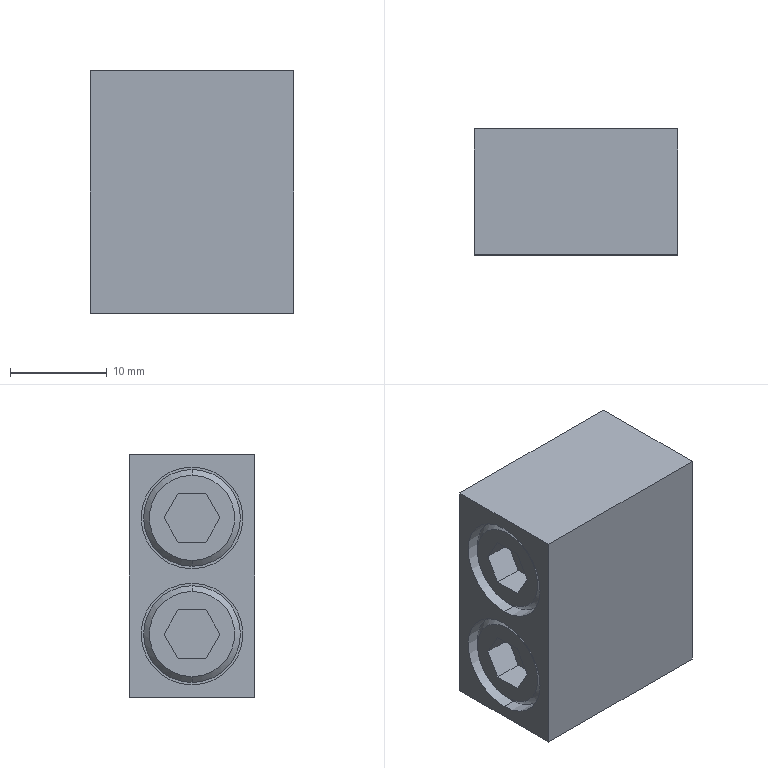Component | SolidWorks | SMC-MXS20-100AS-M9N-1_0SMC-MXS20-100AS-M9N-5-1 | 1 solid | 36 faces | box 21 x 13 x 25 mm | volume 6501 mm3 | plane 24 | cylinder 8 | cone 4 | commonest cylinder face diameters 10 x4 10.5 x4
build123d program:
from build123d import *

# Parameters (mm, degrees)
BOSS_EXTRUDE1_DEPTH      = 6.5
BOSS_EXTRUDE1_DEPTH_BACK = 6.5
SKETCH1_W                = 21
SKETCH1_H                = 25
SKETCH2_R                = 5.25
CUT_EXTRUDE1_DEPTH       = 6.5
SKETCH3_R                = 5.25
CUT_EXTRUDE2_DEPTH       = 6.5
CUT_EXTRUDE3_DEPTH       = 3
CUT_EXTRUDE4_DEPTH       = 3


with BuildPart() as part:
    # Sketch1 → Boss-Extrude1 (new, two sides: drawn at the far end of the back side and taken through both)
    with BuildSketch(Plane(origin=(0, 0, 0), x_dir=(1, 0, 0), z_dir=(0, 1, 0)).offset(-BOSS_EXTRUDE1_DEPTH_BACK)):
        with Locations((-10.5, 0)):
            Rectangle(SKETCH1_W, SKETCH1_H)
    extrude(amount=BOSS_EXTRUDE1_DEPTH + BOSS_EXTRUDE1_DEPTH_BACK)

    # Sketch2 → Cut-Extrude1 (cut)
    with BuildSketch(Plane(origin=(-21, 0, 0), x_dir=(0, 0, -1), z_dir=(1, 0, 0))):
        with Locations((-6, 0)):
            Circle(SKETCH2_R)
    extrude(amount=CUT_EXTRUDE1_DEPTH, mode=Mode.SUBTRACT)

    # Sketch3 → Cut-Extrude2 (cut)
    with BuildSketch(Plane(origin=(-21, 0, 0), x_dir=(0, 0, -1), z_dir=(1, 0, 0))):
        with Locations((6, 0)):
            Circle(SKETCH3_R)
    extrude(amount=CUT_EXTRUDE2_DEPTH, mode=Mode.SUBTRACT)

    # Sketch4 → Revolve1 (revolve)
    with BuildSketch(Plane(origin=(0, 0, 0), x_dir=(1, 0, 0), z_dir=(0, 1, 0)), mode=Mode.PRIVATE) as revolve1_sk:
        Polygon((-14.5, -6), (-14.5, -11), (-19.9, -11), (-20.5, -10.4), (-20.5, -6), align=None)
    revolve(revolve1_sk.sketch.rotate(Axis((-20.5, 0, 6), (1, 0, 0)), 180), axis=Axis((-20.5, 0, 6), (1, 0, 0)))

    # Sketch5 → Revolve2 (revolve)
    with BuildSketch(Plane(origin=(0, 0, 0), x_dir=(1, 0, 0), z_dir=(0, 1, 0)), mode=Mode.PRIVATE) as revolve2_sk:
        Polygon((-14.5, 6), (-14.5, 1), (-19.9, 1), (-20.5, 1.6), (-20.5, 6), align=None)
    revolve(revolve2_sk.sketch.rotate(Axis((-20.5, 0, -6), (1, 0, 0)), 180), axis=Axis((-20.5, 0, -6), (1, 0, 0)))

    # Sketch6 → Cut-Extrude3 (cut)
    with BuildSketch(Plane(origin=(-20.5, 0, 0), x_dir=(0, 0, -1), z_dir=(1, 0, 0))):
        Polygon((-8.5, 1.443), (-8.5, -1.443), (-6, -2.887), (-3.5, -1.443), (-3.5, 1.443), (-6, 2.887), align=None)
    extrude(amount=CUT_EXTRUDE3_DEPTH, mode=Mode.SUBTRACT)

    # Sketch7 → Cut-Extrude4 (cut)
    with BuildSketch(Plane(origin=(-20.5, 0, 0), x_dir=(0, 0, -1), z_dir=(1, 0, 0))):
        Polygon((3.5, 1.443), (3.5, -1.443), (6, -2.887), (8.5, -1.443), (8.5, 1.443), (6, 2.887), align=None)
    extrude(amount=CUT_EXTRUDE4_DEPTH, mode=Mode.SUBTRACT)


solid = part.part

# Placed as in the assembly
solid = solid.moved(Location((-271.009, 86.721, 82.589), (0, 0, 0)))
STEP:
#1=COLOUR_RGB('',0.7922,0.8196,0.9333);
#2=FILL_AREA_STYLE_COLOUR('',#1);
#3=FILL_AREA_STYLE('',(#2));
#4=SURFACE_STYLE_FILL_AREA(#3);
#5=SURFACE_SIDE_STYLE('',(#4));
#6=SURFACE_STYLE_USAGE(.BOTH.,#5);
#7=PRESENTATION_STYLE_ASSIGNMENT((#6));
#8=CARTESIAN_POINT('',(-11.477,3.414,2.842));
#9=VERTEX_POINT('',#8);
#10=CARTESIAN_POINT('',(-11.477,3.414,3.189));
#11=VERTEX_POINT('',#10);
#12=CARTESIAN_POINT('',(-11.477,3.414,3.015));
#13=DIRECTION('',(1.,0.,0.));
#14=DIRECTION('',(0.,0.,-1.));
#15=AXIS2_PLACEMENT_3D('',#12,#13,#14);
#16=CIRCLE('',#15,0.1732);
#17=EDGE_CURVE('',#9,#11,#16,.T.);
#18=ORIENTED_EDGE('',*,*,#17,.T.);
#19=CARTESIAN_POINT('',(-11.453,3.414,3.212));
#20=VERTEX_POINT('',#19);
#21=CARTESIAN_POINT('',(-11.477,3.414,3.189));
#22=DIRECTION('',(0.7071,0.,0.7071));
#23=VECTOR('',#22,39.37);
#24=LINE('',#21,#23);
#25=EDGE_CURVE('',#11,#20,#24,.T.);
#26=ORIENTED_EDGE('',*,*,#25,.T.);
#27=CARTESIAN_POINT('',(-11.453,3.414,2.818));
#28=VERTEX_POINT('',#27);
#29=CARTESIAN_POINT('',(-11.453,3.414,3.015));
#30=DIRECTION('',(1.,0.,0.));
#31=DIRECTION('',(0.,0.,-1.));
#32=AXIS2_PLACEMENT_3D('',#29,#30,#31);
#33=CIRCLE('',#32,0.1969);
#34=EDGE_CURVE('',#28,#20,#33,.T.);
#35=ORIENTED_EDGE('',*,*,#34,.F.);
#36=CARTESIAN_POINT('',(-11.477,3.414,2.842));
#37=DIRECTION('',(0.7071,0.,-0.7071));
#38=VECTOR('',#37,39.37);
#39=LINE('',#36,#38);
#40=EDGE_CURVE('',#9,#28,#39,.T.);
#41=ORIENTED_EDGE('',*,*,#40,.F.);
#42=EDGE_LOOP('',(#18,#26,#35,#41));
#43=FACE_OUTER_BOUND('',#42,.T.);
#44=CARTESIAN_POINT('',(-11.477,3.414,3.015));
#45=DIRECTION('',(1.,0.,0.));
#46=DIRECTION('',(0.,0.,-1.));
#47=AXIS2_PLACEMENT_3D('',#44,#45,#46);
#48=CONICAL_SURFACE('',#47,0.1732,0.7854);
#49=ADVANCED_FACE('',(#43),#48,.T.);
#50=ORIENTED_EDGE('',*,*,#34,.T.);
#51=CARTESIAN_POINT('',(-11.241,3.414,3.212));
#52=VERTEX_POINT('',#51);
#53=CARTESIAN_POINT('',(-11.477,3.414,3.212));
#54=DIRECTION('',(1.,0.,0.));
#55=VECTOR('',#54,39.37);
#56=LINE('',#53,#55);
#57=EDGE_CURVE('',#20,#52,#56,.T.);
#58=ORIENTED_EDGE('',*,*,#57,.T.);
#59=CARTESIAN_POINT('',(-11.241,3.414,2.818));
#60=VERTEX_POINT('',#59);
#61=CARTESIAN_POINT('',(-11.241,3.414,3.015));
#62=DIRECTION('',(-1.,0.,0.));
#63=DIRECTION('',(0.,0.,-1.));
#64=AXIS2_PLACEMENT_3D('',#61,#62,#63);
#65=CIRCLE('',#64,0.1969);
#66=EDGE_CURVE('',#52,#60,#65,.T.);
#67=ORIENTED_EDGE('',*,*,#66,.T.);
#68=CARTESIAN_POINT('',(-11.477,3.414,2.818));
#69=DIRECTION('',(1.,0.,0.));
#70=VECTOR('',#69,39.37);
#71=LINE('',#68,#70);
#72=EDGE_CURVE('',#28,#60,#71,.T.);
#73=ORIENTED_EDGE('',*,*,#72,.F.);
#74=EDGE_LOOP('',(#50,#58,#67,#73));
#75=FACE_OUTER_BOUND('',#74,.T.);
#76=CARTESIAN_POINT('',(-11.477,3.414,3.015));
#77=DIRECTION('',(1.,0.,0.));
#78=DIRECTION('',(0.,0.,-1.));
#79=AXIS2_PLACEMENT_3D('',#76,#77,#78);
#80=CYLINDRICAL_SURFACE('',#79,0.1969);
#81=ADVANCED_FACE('',(#75),#80,.T.);
#82=CARTESIAN_POINT('',(-11.477,3.414,3.315));
#83=VERTEX_POINT('',#82);
#84=CARTESIAN_POINT('',(-11.477,3.414,3.661));
#85=VERTEX_POINT('',#84);
#86=CARTESIAN_POINT('',(-11.477,3.414,3.488));
#87=DIRECTION('',(1.,0.,0.));
#88=DIRECTION('',(0.,0.,-1.));
#89=AXIS2_PLACEMENT_3D('',#86,#87,#88);
#90=CIRCLE('',#89,0.1732);
#91=EDGE_CURVE('',#83,#85,#90,.T.);
#92=ORIENTED_EDGE('',*,*,#91,.T.);
#93=CARTESIAN_POINT('',(-11.453,3.414,3.685));
#94=VERTEX_POINT('',#93);
#95=CARTESIAN_POINT('',(-11.477,3.414,3.661));
#96=DIRECTION('',(0.7071,0.,0.7071));
#97=VECTOR('',#96,39.37);
#98=LINE('',#95,#97);
#99=EDGE_CURVE('',#85,#94,#98,.T.);
#100=ORIENTED_EDGE('',*,*,#99,.T.);
#101=CARTESIAN_POINT('',(-11.453,3.414,3.291));
#102=VERTEX_POINT('',#101);
#103=CARTESIAN_POINT('',(-11.453,3.414,3.488));
#104=DIRECTION('',(1.,0.,0.));
#105=DIRECTION('',(0.,0.,-1.));
#106=AXIS2_PLACEMENT_3D('',#103,#104,#105);
#107=CIRCLE('',#106,0.1969);
#108=EDGE_CURVE('',#102,#94,#107,.T.);
#109=ORIENTED_EDGE('',*,*,#108,.F.);
#110=CARTESIAN_POINT('',(-11.477,3.414,3.315));
#111=DIRECTION('',(0.7071,0.,-0.7071));
#112=VECTOR('',#111,39.37);
#113=LINE('',#110,#112);
#114=EDGE_CURVE('',#83,#102,#113,.T.);
#115=ORIENTED_EDGE('',*,*,#114,.F.);
#116=EDGE_LOOP('',(#92,#100,#109,#115));
#117=FACE_OUTER_BOUND('',#116,.T.);
#118=CARTESIAN_POINT('',(-11.477,3.414,3.488));
#119=DIRECTION('',(1.,0.,0.));
#120=DIRECTION('',(0.,0.,-1.));
#121=AXIS2_PLACEMENT_3D('',#118,#119,#120);
#122=CONICAL_SURFACE('',#121,0.1732,0.7854);
#123=ADVANCED_FACE('',(#117),#122,.T.);
#124=ORIENTED_EDGE('',*,*,#108,.T.);
#125=CARTESIAN_POINT('',(-11.241,3.414,3.685));
#126=VERTEX_POINT('',#125);
#127=CARTESIAN_POINT('',(-11.477,3.414,3.685));
#128=DIRECTION('',(1.,0.,0.));
#129=VECTOR('',#128,39.37);
#130=LINE('',#127,#129);
#131=EDGE_CURVE('',#94,#126,#130,.T.);
#132=ORIENTED_EDGE('',*,*,#131,.T.);
#133=CARTESIAN_POINT('',(-11.241,3.414,3.291));
#134=VERTEX_POINT('',#133);
#135=CARTESIAN_POINT('',(-11.241,3.414,3.488));
#136=DIRECTION('',(-1.,0.,0.));
#137=DIRECTION('',(0.,0.,-1.));
#138=AXIS2_PLACEMENT_3D('',#135,#136,#137);
#139=CIRCLE('',#138,0.1969);
#140=EDGE_CURVE('',#126,#134,#139,.T.);
#141=ORIENTED_EDGE('',*,*,#140,.T.);
#142=CARTESIAN_POINT('',(-11.477,3.414,3.291));
#143=DIRECTION('',(1.,0.,0.));
#144=VECTOR('',#143,39.37);
#145=LINE('',#142,#144);
#146=EDGE_CURVE('',#102,#134,#145,.T.);
#147=ORIENTED_EDGE('',*,*,#146,.F.);
#148=EDGE_LOOP('',(#124,#132,#141,#147));
#149=FACE_OUTER_BOUND('',#148,.T.);
#150=CARTESIAN_POINT('',(-11.477,3.414,3.488));
#151=DIRECTION('',(1.,0.,0.));
#152=DIRECTION('',(0.,0.,-1.));
#153=AXIS2_PLACEMENT_3D('',#150,#151,#152);
#154=CYLINDRICAL_SURFACE('',#153,0.1969);
#155=ADVANCED_FACE('',(#149),#154,.T.);
#156=CARTESIAN_POINT('',(-11.241,3.414,3.222));
#157=VERTEX_POINT('',#156);
#158=CARTESIAN_POINT('',(-11.241,3.414,2.809));
#159=VERTEX_POINT('',#158);
#160=CARTESIAN_POINT('',(-11.241,3.414,3.015));
#161=DIRECTION('',(1.,0.,0.));
#162=DIRECTION('',(0.,0.,-1.));
#163=AXIS2_PLACEMENT_3D('',#160,#161,#162);
#164=CIRCLE('',#163,0.2067);
#165=EDGE_CURVE('',#157,#159,#164,.T.);
#166=ORIENTED_EDGE('',*,*,#165,.T.);
#167=CARTESIAN_POINT('',(-11.496,3.414,2.809));
#168=VERTEX_POINT('',#167);
#169=CARTESIAN_POINT('',(-11.241,3.414,2.809));
#170=DIRECTION('',(-1.,0.,0.));
#171=VECTOR('',#170,39.37);
#172=LINE('',#169,#171);
#173=EDGE_CURVE('',#159,#168,#172,.T.);
#174=ORIENTED_EDGE('',*,*,#173,.T.);
#175=CARTESIAN_POINT('',(-11.496,3.414,3.222));
#176=VERTEX_POINT('',#175);
#177=CARTESIAN_POINT('',(-11.496,3.414,3.015));
#178=DIRECTION('',(1.,0.,0.));
#179=DIRECTION('',(0.,0.,-1.));
#180=AXIS2_PLACEMENT_3D('',#177,#178,#179);
#181=CIRCLE('',#180,0.2067);
#182=EDGE_CURVE('',#176,#168,#181,.T.);
#183=ORIENTED_EDGE('',*,*,#182,.F.);
#184=CARTESIAN_POINT('',(-11.241,3.414,3.222));
#185=DIRECTION('',(-1.,0.,0.));
#186=VECTOR('',#185,39.37);
#187=LINE('',#184,#186);
#188=EDGE_CURVE('',#157,#176,#187,.T.);
#189=ORIENTED_EDGE('',*,*,#188,.F.);
#190=EDGE_LOOP('',(#166,#174,#183,#189));
#191=FACE_OUTER_BOUND('',#190,.T.);
#192=CARTESIAN_POINT('',(-11.241,3.414,3.015));
#193=DIRECTION('',(-1.,0.,0.));
#194=DIRECTION('',(0.,0.,1.));
#195=AXIS2_PLACEMENT_3D('',#192,#193,#194);
#196=CYLINDRICAL_SURFACE('',#195,0.2067);
#197=ADVANCED_FACE('',(#191),#196,.F.);
#198=CARTESIAN_POINT('',(-11.241,3.414,3.694));
#199=VERTEX_POINT('',#198);
#200=CARTESIAN_POINT('',(-11.241,3.414,3.281));
#201=VERTEX_POINT('',#200);
#202=CARTESIAN_POINT('',(-11.241,3.414,3.488));
#203=DIRECTION('',(1.,0.,0.));
#204=DIRECTION('',(0.,0.,-1.));
#205=AXIS2_PLACEMENT_3D('',#202,#203,#204);
#206=CIRCLE('',#205,0.2067);
#207=EDGE_CURVE('',#199,#201,#206,.T.);
#208=ORIENTED_EDGE('',*,*,#207,.T.);
#209=CARTESIAN_POINT('',(-11.496,3.414,3.281));
#210=VERTEX_POINT('',#209);
#211=CARTESIAN_POINT('',(-11.241,3.414,3.281));
#212=DIRECTION('',(-1.,0.,0.));
#213=VECTOR('',#212,39.37);
#214=LINE('',#211,#213);
#215=EDGE_CURVE('',#201,#210,#214,.T.);
#216=ORIENTED_EDGE('',*,*,#215,.T.);
#217=CARTESIAN_POINT('',(-11.496,3.414,3.694));
#218=VERTEX_POINT('',#217);
#219=CARTESIAN_POINT('',(-11.496,3.414,3.488));
#220=DIRECTION('',(1.,0.,0.));
#221=DIRECTION('',(0.,0.,-1.));
#222=AXIS2_PLACEMENT_3D('',#219,#220,#221);
#223=CIRCLE('',#222,0.2067);
#224=EDGE_CURVE('',#218,#210,#223,.T.);
#225=ORIENTED_EDGE('',*,*,#224,.F.);
#226=CARTESIAN_POINT('',(-11.241,3.414,3.694));
#227=DIRECTION('',(-1.,0.,0.));
#228=VECTOR('',#227,39.37);
#229=LINE('',#226,#228);
#230=EDGE_CURVE('',#199,#218,#229,.T.);
#231=ORIENTED_EDGE('',*,*,#230,.F.);
#232=EDGE_LOOP('',(#208,#216,#225,#231));
#233=FACE_OUTER_BOUND('',#232,.T.);
#234=CARTESIAN_POINT('',(-11.241,3.414,3.488));
#235=DIRECTION('',(-1.,0.,0.));
#236=DIRECTION('',(0.,0.,1.));
#237=AXIS2_PLACEMENT_3D('',#234,#235,#236);
#238=CYLINDRICAL_SURFACE('',#237,0.2067);
#239=ADVANCED_FACE('',(#233),#238,.F.);
#240=ORIENTED_EDGE('',*,*,#17,.F.);
#241=CARTESIAN_POINT('',(-11.477,3.414,3.015));
#242=DIRECTION('',(1.,0.,0.));
#243=DIRECTION('',(0.,0.,-1.));
#244=AXIS2_PLACEMENT_3D('',#241,#242,#243);
#245=CIRCLE('',#244,0.1732);
#246=EDGE_CURVE('',#11,#9,#245,.T.);
#247=ORIENTED_EDGE('',*,*,#246,.F.);
#248=EDGE_LOOP('',(#240,#247));
#249=FACE_OUTER_BOUND('',#248,.T.);
#250=CARTESIAN_POINT('',(-11.477,3.528,3.015));
#251=VERTEX_POINT('',#250);
#252=CARTESIAN_POINT('',(-11.477,3.471,3.114));
#253=VERTEX_POINT('',#252);
#254=CARTESIAN_POINT('',(-11.477,3.528,3.015));
#255=DIRECTION('',(0.,-0.5,0.866));
#256=VECTOR('',#255,39.37);
#257=LINE('',#254,#256);
#258=EDGE_CURVE('',#251,#253,#257,.T.);
#259=ORIENTED_EDGE('',*,*,#258,.T.);
#260=CARTESIAN_POINT('',(-11.477,3.357,3.114));
#261=VERTEX_POINT('',#260);
#262=CARTESIAN_POINT('',(-11.477,3.471,3.114));
#263=DIRECTION('',(0.,-1.,0.));
#264=VECTOR('',#263,39.37);
#265=LINE('',#262,#264);
#266=EDGE_CURVE('',#253,#261,#265,.T.);
#267=ORIENTED_EDGE('',*,*,#266,.T.);
#268=CARTESIAN_POINT('',(-11.477,3.301,3.015));
#269=VERTEX_POINT('',#268);
#270=CARTESIAN_POINT('',(-11.477,3.357,3.114));
#271=DIRECTION('',(0.,-0.5,-0.866));
#272=VECTOR('',#271,39.37);
#273=LINE('',#270,#272);
#274=EDGE_CURVE('',#261,#269,#273,.T.);
#275=ORIENTED_EDGE('',*,*,#274,.T.);
#276=CARTESIAN_POINT('',(-11.477,3.357,2.917));
#277=VERTEX_POINT('',#276);
#278=CARTESIAN_POINT('',(-11.477,3.301,3.015));
#279=DIRECTION('',(0.,0.5,-0.866));
#280=VECTOR('',#279,39.37);
#281=LINE('',#278,#280);
#282=EDGE_CURVE('',#269,#277,#281,.T.);
#283=ORIENTED_EDGE('',*,*,#282,.T.);
#284=CARTESIAN_POINT('',(-11.477,3.471,2.917));
#285=VERTEX_POINT('',#284);
#286=CARTESIAN_POINT('',(-11.477,3.357,2.917));
#287=DIRECTION('',(0.,1.,0.));
#288=VECTOR('',#287,39.37);
#289=LINE('',#286,#288);
#290=EDGE_CURVE('',#277,#285,#289,.T.);
#291=ORIENTED_EDGE('',*,*,#290,.T.);
#292=CARTESIAN_POINT('',(-11.477,3.471,2.917));
#293=DIRECTION('',(0.,0.5,0.866));
#294=VECTOR('',#293,39.37);
#295=LINE('',#292,#294);
#296=EDGE_CURVE('',#285,#251,#295,.T.);
#297=ORIENTED_EDGE('',*,*,#296,.T.);
#298=EDGE_LOOP('',(#259,#267,#275,#283,#291,#297));
#299=FACE_BOUND('',#298,.T.);
#300=CARTESIAN_POINT('',(-11.477,3.414,3.189));
#301=DIRECTION('',(1.,0.,0.));
#302=DIRECTION('',(0.,0.,-1.));
#303=AXIS2_PLACEMENT_3D('',#300,#301,#302);
#304=PLANE('',#303);
#305=ADVANCED_FACE('',(#249,#299),#304,.F.);
#306=ORIENTED_EDGE('',*,*,#91,.F.);
#307=CARTESIAN_POINT('',(-11.477,3.414,3.488));
#308=DIRECTION('',(1.,0.,0.));
#309=DIRECTION('',(0.,0.,-1.));
#310=AXIS2_PLACEMENT_3D('',#307,#308,#309);
#311=CIRCLE('',#310,0.1732);
#312=EDGE_CURVE('',#85,#83,#311,.T.);
#313=ORIENTED_EDGE('',*,*,#312,.F.);
#314=EDGE_LOOP('',(#306,#313));
#315=FACE_OUTER_BOUND('',#314,.T.);
#316=CARTESIAN_POINT('',(-11.477,3.528,3.488));
#317=VERTEX_POINT('',#316);
#318=CARTESIAN_POINT('',(-11.477,3.471,3.586));
#319=VERTEX_POINT('',#318);
#320=CARTESIAN_POINT('',(-11.477,3.528,3.488));
#321=DIRECTION('',(0.,-0.5,0.866));
#322=VECTOR('',#321,39.37);
#323=LINE('',#320,#322);
#324=EDGE_CURVE('',#317,#319,#323,.T.);
#325=ORIENTED_EDGE('',*,*,#324,.T.);
#326=CARTESIAN_POINT('',(-11.477,3.357,3.586));
#327=VERTEX_POINT('',#326);
#328=CARTESIAN_POINT('',(-11.477,3.471,3.586));
#329=DIRECTION('',(0.,-1.,0.));
#330=VECTOR('',#329,39.37);
#331=LINE('',#328,#330);
#332=EDGE_CURVE('',#319,#327,#331,.T.);
#333=ORIENTED_EDGE('',*,*,#332,.T.);
#334=CARTESIAN_POINT('',(-11.477,3.301,3.488));
#335=VERTEX_POINT('',#334);
#336=CARTESIAN_POINT('',(-11.477,3.357,3.586));
#337=DIRECTION('',(0.,-0.5,-0.866));
#338=VECTOR('',#337,39.37);
#339=LINE('',#336,#338);
#340=EDGE_CURVE('',#327,#335,#339,.T.);
#341=ORIENTED_EDGE('',*,*,#340,.T.);
#342=CARTESIAN_POINT('',(-11.477,3.357,3.389));
#343=VERTEX_POINT('',#342);
#344=CARTESIAN_POINT('',(-11.477,3.301,3.488));
#345=DIRECTION('',(0.,0.5,-0.866));
#346=VECTOR('',#345,39.37);
#347=LINE('',#344,#346);
#348=EDGE_CURVE('',#335,#343,#347,.T.);
#349=ORIENTED_EDGE('',*,*,#348,.T.);
#350=CARTESIAN_POINT('',(-11.477,3.471,3.389));
#351=VERTEX_POINT('',#350);
#352=CARTESIAN_POINT('',(-11.477,3.357,3.389));
#353=DIRECTION('',(0.,1.,0.));
#354=VECTOR('',#353,39.37);
#355=LINE('',#352,#354);
#356=EDGE_CURVE('',#343,#351,#355,.T.);
#357=ORIENTED_EDGE('',*,*,#356,.T.);
#358=CARTESIAN_POINT('',(-11.477,3.471,3.389));
#359=DIRECTION('',(0.,0.5,0.866));
#360=VECTOR('',#359,39.37);
#361=LINE('',#358,#360);
#362=EDGE_CURVE('',#351,#317,#361,.T.);
#363=ORIENTED_EDGE('',*,*,#362,.T.);
#364=EDGE_LOOP('',(#325,#333,#341,#349,#357,#363));
#365=FACE_BOUND('',#364,.T.);
#366=CARTESIAN_POINT('',(-11.477,3.414,3.661));
#367=DIRECTION('',(1.,0.,0.));
#368=DIRECTION('',(0.,0.,-1.));
#369=AXIS2_PLACEMENT_3D('',#366,#367,#368);
#370=PLANE('',#369);
#371=ADVANCED_FACE('',(#315,#365),#370,.F.);
#372=ORIENTED_EDGE('',*,*,#165,.F.);
#373=CARTESIAN_POINT('',(-11.241,3.414,3.015));
#374=DIRECTION('',(1.,0.,0.));
#375=DIRECTION('',(0.,0.,-1.));
#376=AXIS2_PLACEMENT_3D('',#373,#374,#375);
#377=CIRCLE('',#376,0.2067);
#378=EDGE_CURVE('',#159,#157,#377,.T.);
#379=ORIENTED_EDGE('',*,*,#378,.F.);
#380=EDGE_LOOP('',(#372,#379));
#381=FACE_OUTER_BOUND('',#380,.T.);
#382=CARTESIAN_POINT('',(-11.241,3.414,3.015));
#383=DIRECTION('',(-1.,0.,0.));
#384=DIRECTION('',(0.,0.,-1.));
#385=AXIS2_PLACEMENT_3D('',#382,#383,#384);
#386=CIRCLE('',#385,0.1969);
#387=EDGE_CURVE('',#60,#52,#386,.T.);
#388=ORIENTED_EDGE('',*,*,#387,.F.);
#389=ORIENTED_EDGE('',*,*,#66,.F.);
#390=EDGE_LOOP('',(#388,#389));
#391=FACE_BOUND('',#390,.T.);
#392=CARTESIAN_POINT('',(-11.241,3.414,3.015));
#393=DIRECTION('',(1.,0.,0.));
#394=DIRECTION('',(0.,0.,-1.));
#395=AXIS2_PLACEMENT_3D('',#392,#393,#394);
#396=PLANE('',#395);
#397=ADVANCED_FACE('',(#381,#391),#396,.F.);
#398=ORIENTED_EDGE('',*,*,#207,.F.);
#399=CARTESIAN_POINT('',(-11.241,3.414,3.488));
#400=DIRECTION('',(1.,0.,0.));
#401=DIRECTION('',(0.,0.,-1.));
#402=AXIS2_PLACEMENT_3D('',#399,#400,#401);
#403=CIRCLE('',#402,0.2067);
#404=EDGE_CURVE('',#201,#199,#403,.T.);
#405=ORIENTED_EDGE('',*,*,#404,.F.);
#406=EDGE_LOOP('',(#398,#405));
#407=FACE_OUTER_BOUND('',#406,.T.);
#408=CARTESIAN_POINT('',(-11.241,3.414,3.488));
#409=DIRECTION('',(-1.,0.,0.));
#410=DIRECTION('',(0.,0.,-1.));
#411=AXIS2_PLACEMENT_3D('',#408,#409,#410);
#412=CIRCLE('',#411,0.1969);
#413=EDGE_CURVE('',#134,#126,#412,.T.);
#414=ORIENTED_EDGE('',*,*,#413,.F.);
#415=ORIENTED_EDGE('',*,*,#140,.F.);
#416=EDGE_LOOP('',(#414,#415));
#417=FACE_BOUND('',#416,.T.);
#418=CARTESIAN_POINT('',(-11.241,3.414,3.488));
#419=DIRECTION('',(1.,0.,0.));
#420=DIRECTION('',(0.,0.,-1.));
#421=AXIS2_PLACEMENT_3D('',#418,#419,#420);
#422=PLANE('',#421);
#423=ADVANCED_FACE('',(#407,#417),#422,.F.);
#424=ORIENTED_EDGE('',*,*,#224,.T.);
#425=CARTESIAN_POINT('',(-11.496,3.414,3.488));
#426=DIRECTION('',(1.,0.,0.));
#427=DIRECTION('',(0.,0.,-1.));
#428=AXIS2_PLACEMENT_3D('',#425,#426,#427);
#429=CIRCLE('',#428,0.2067);
#430=EDGE_CURVE('',#210,#218,#429,.T.);
#431=ORIENTED_EDGE('',*,*,#430,.T.);
#432=EDGE_LOOP('',(#424,#431));
#433=FACE_BOUND('',#432,.T.);
#434=CARTESIAN_POINT('',(-11.496,3.67,2.759));
#435=VERTEX_POINT('',#434);
#436=CARTESIAN_POINT('',(-11.496,3.158,2.759));
#437=VERTEX_POINT('',#436);
#438=CARTESIAN_POINT('',(-11.496,3.67,2.759));
#439=DIRECTION('',(0.,-1.,0.));
#440=VECTOR('',#439,39.37);
#441=LINE('',#438,#440);
#442=EDGE_CURVE('',#435,#437,#441,.T.);
#443=ORIENTED_EDGE('',*,*,#442,.T.);
#444=CARTESIAN_POINT('',(-11.496,3.158,3.744));
#445=VERTEX_POINT('',#444);
#446=CARTESIAN_POINT('',(-11.496,3.158,2.759));
#447=DIRECTION('',(0.,0.,1.));
#448=VECTOR('',#447,39.37);
#449=LINE('',#446,#448);
#450=EDGE_CURVE('',#437,#445,#449,.T.);
#451=ORIENTED_EDGE('',*,*,#450,.T.);
#452=CARTESIAN_POINT('',(-11.496,3.67,3.744));
#453=VERTEX_POINT('',#452);
#454=CARTESIAN_POINT('',(-11.496,3.67,3.744));
#455=DIRECTION('',(0.,-1.,0.));
#456=VECTOR('',#455,39.37);
#457=LINE('',#454,#456);
#458=EDGE_CURVE('',#453,#445,#457,.T.);
#459=ORIENTED_EDGE('',*,*,#458,.F.);
#460=CARTESIAN_POINT('',(-11.496,3.67,2.759));
#461=DIRECTION('',(0.,0.,1.));
#462=VECTOR('',#461,39.37);
#463=LINE('',#460,#462);
#464=EDGE_CURVE('',#435,#453,#463,.T.);
#465=ORIENTED_EDGE('',*,*,#464,.F.);
#466=EDGE_LOOP('',(#443,#451,#459,#465));
#467=FACE_OUTER_BOUND('',#466,.T.);
#468=ORIENTED_EDGE('',*,*,#182,.T.);
#469=CARTESIAN_POINT('',(-11.496,3.414,3.015));
#470=DIRECTION('',(1.,0.,0.));
#471=DIRECTION('',(0.,0.,-1.));
#472=AXIS2_PLACEMENT_3D('',#469,#470,#471);
#473=CIRCLE('',#472,0.2067);
#474=EDGE_CURVE('',#168,#176,#473,.T.);
#475=ORIENTED_EDGE('',*,*,#474,.T.);
#476=EDGE_LOOP('',(#468,#475));
#477=FACE_BOUND('',#476,.T.);
#478=CARTESIAN_POINT('',(-11.496,3.67,2.759));
#479=DIRECTION('',(1.,0.,0.));
#480=DIRECTION('',(0.,0.,-1.));
#481=AXIS2_PLACEMENT_3D('',#478,#479,#480);
#482=PLANE('',#481);
#483=ADVANCED_FACE('',(#433,#467,#477),#482,.F.);
#484=ORIENTED_EDGE('',*,*,#458,.T.);
#485=CARTESIAN_POINT('',(-10.67,3.158,3.744));
#486=VERTEX_POINT('',#485);
#487=CARTESIAN_POINT('',(-11.496,3.158,3.744));
#488=DIRECTION('',(1.,0.,0.));
#489=VECTOR('',#488,39.37);
#490=LINE('',#487,#489);
#491=EDGE_CURVE('',#445,#486,#490,.T.);
#492=ORIENTED_EDGE('',*,*,#491,.T.);
#493=CARTESIAN_POINT('',(-10.67,3.67,3.744));
#494=VERTEX_POINT('',#493);
#495=CARTESIAN_POINT('',(-10.67,3.67,3.744));
#496=DIRECTION('',(0.,-1.,0.));
#497=VECTOR('',#496,39.37);
#498=LINE('',#495,#497);
#499=EDGE_CURVE('',#494,#486,#498,.T.);
#500=ORIENTED_EDGE('',*,*,#499,.F.);
#501=CARTESIAN_POINT('',(-11.496,3.67,3.744));
#502=DIRECTION('',(1.,0.,0.));
#503=VECTOR('',#502,39.37);
#504=LINE('',#501,#503);
#505=EDGE_CURVE('',#453,#494,#504,.T.);
#506=ORIENTED_EDGE('',*,*,#505,.F.);
#507=EDGE_LOOP('',(#484,#492,#500,#506));
#508=FACE_OUTER_BOUND('',#507,.T.);
#509=CARTESIAN_POINT('',(-11.496,3.67,3.744));
#510=DIRECTION('',(0.,0.,-1.));
#511=DIRECTION('',(-1.,0.,0.));
#512=AXIS2_PLACEMENT_3D('',#509,#510,#511);
#513=PLANE('',#512);
#514=ADVANCED_FACE('',(#508),#513,.F.);
#515=ORIENTED_EDGE('',*,*,#499,.T.);
#516=CARTESIAN_POINT('',(-10.67,3.158,2.759));
#517=VERTEX_POINT('',#516);
#518=CARTESIAN_POINT('',(-10.67,3.158,3.744));
#519=DIRECTION('',(0.,0.,-1.));
#520=VECTOR('',#519,39.37);
#521=LINE('',#518,#520);
#522=EDGE_CURVE('',#486,#517,#521,.T.);
#523=ORIENTED_EDGE('',*,*,#522,.T.);
#524=CARTESIAN_POINT('',(-10.67,3.67,2.759));
#525=VERTEX_POINT('',#524);
#526=CARTESIAN_POINT('',(-10.67,3.67,2.759));
#527=DIRECTION('',(0.,-1.,0.));
#528=VECTOR('',#527,39.37);
#529=LINE('',#526,#528);
#530=EDGE_CURVE('',#525,#517,#529,.T.);
#531=ORIENTED_EDGE('',*,*,#530,.F.);
#532=CARTESIAN_POINT('',(-10.67,3.67,3.744));
#533=DIRECTION('',(0.,0.,-1.));
#534=VECTOR('',#533,39.37);
#535=LINE('',#532,#534);
#536=EDGE_CURVE('',#494,#525,#535,.T.);
#537=ORIENTED_EDGE('',*,*,#536,.F.);
#538=EDGE_LOOP('',(#515,#523,#531,#537));
#539=FACE_OUTER_BOUND('',#538,.T.);
#540=CARTESIAN_POINT('',(-10.67,3.67,3.744));
#541=DIRECTION('',(-1.,0.,0.));
#542=DIRECTION('',(0.,0.,1.));
#543=AXIS2_PLACEMENT_3D('',#540,#541,#542);
#544=PLANE('',#543);
#545=ADVANCED_FACE('',(#539),#544,.F.);
#546=ORIENTED_EDGE('',*,*,#530,.T.);
#547=CARTESIAN_POINT('',(-10.67,3.158,2.759));
#548=DIRECTION('',(-1.,0.,0.));
#549=VECTOR('',#548,39.37);
#550=LINE('',#547,#549);
#551=EDGE_CURVE('',#517,#437,#550,.T.);
#552=ORIENTED_EDGE('',*,*,#551,.T.);
#553=ORIENTED_EDGE('',*,*,#442,.F.);
#554=CARTESIAN_POINT('',(-10.67,3.67,2.759));
#555=DIRECTION('',(-1.,0.,0.));
#556=VECTOR('',#555,39.37);
#557=LINE('',#554,#556);
#558=EDGE_CURVE('',#525,#435,#557,.T.);
#559=ORIENTED_EDGE('',*,*,#558,.F.);
#560=EDGE_LOOP('',(#546,#552,#553,#559));
#561=FACE_OUTER_BOUND('',#560,.T.);
#562=CARTESIAN_POINT('',(-10.67,3.67,2.759));
#563=DIRECTION('',(0.,0.,1.));
#564=DIRECTION('',(1.,0.,0.));
#565=AXIS2_PLACEMENT_3D('',#562,#563,#564);
#566=PLANE('',#565);
#567=ADVANCED_FACE('',(#561),#566,.F.);
#568=ORIENTED_EDGE('',*,*,#464,.T.);
#569=ORIENTED_EDGE('',*,*,#505,.T.);
#570=ORIENTED_EDGE('',*,*,#536,.T.);
#571=ORIENTED_EDGE('',*,*,#558,.T.);
#572=EDGE_LOOP('',(#568,#569,#570,#571));
#573=FACE_OUTER_BOUND('',#572,.T.);
#574=CARTESIAN_POINT('',(-10.67,3.67,3.252));
#575=DIRECTION('',(0.,1.,0.));
#576=DIRECTION('',(0.,0.,1.));
#577=AXIS2_PLACEMENT_3D('',#574,#575,#576);
#578=PLANE('',#577);
#579=ADVANCED_FACE('',(#573),#578,.T.);
#580=ORIENTED_EDGE('',*,*,#450,.F.);
#581=ORIENTED_EDGE('',*,*,#551,.F.);
#582=ORIENTED_EDGE('',*,*,#522,.F.);
#583=ORIENTED_EDGE('',*,*,#491,.F.);
#584=EDGE_LOOP('',(#580,#581,#582,#583));
#585=FACE_OUTER_BOUND('',#584,.T.);
#586=CARTESIAN_POINT('',(-10.67,3.158,3.252));
#587=DIRECTION('',(0.,1.,0.));
#588=DIRECTION('',(0.,0.,1.));
#589=AXIS2_PLACEMENT_3D('',#586,#587,#588);
#590=PLANE('',#589);
#591=ADVANCED_FACE('',(#585),#590,.F.);
#592=ORIENTED_EDGE('',*,*,#215,.F.);
#593=ORIENTED_EDGE('',*,*,#404,.T.);
#594=ORIENTED_EDGE('',*,*,#230,.T.);
#595=ORIENTED_EDGE('',*,*,#430,.F.);
#596=EDGE_LOOP('',(#592,#593,#594,#595));
#597=FACE_OUTER_BOUND('',#596,.T.);
#598=CARTESIAN_POINT('',(-11.241,3.414,3.488));
#599=DIRECTION('',(-1.,0.,0.));
#600=DIRECTION('',(0.,0.,1.));
#601=AXIS2_PLACEMENT_3D('',#598,#599,#600);
#602=CYLINDRICAL_SURFACE('',#601,0.2067);
#603=ADVANCED_FACE('',(#597),#602,.F.);
#604=ORIENTED_EDGE('',*,*,#173,.F.);
#605=ORIENTED_EDGE('',*,*,#378,.T.);
#606=ORIENTED_EDGE('',*,*,#188,.T.);
#607=ORIENTED_EDGE('',*,*,#474,.F.);
#608=EDGE_LOOP('',(#604,#605,#606,#607));
#609=FACE_OUTER_BOUND('',#608,.T.);
#610=CARTESIAN_POINT('',(-11.241,3.414,3.015));
#611=DIRECTION('',(-1.,0.,0.));
#612=DIRECTION('',(0.,0.,1.));
#613=AXIS2_PLACEMENT_3D('',#610,#611,#612);
#614=CYLINDRICAL_SURFACE('',#613,0.2067);
#615=ADVANCED_FACE('',(#609),#614,.F.);
#616=ORIENTED_EDGE('',*,*,#131,.F.);
#617=CARTESIAN_POINT('',(-11.453,3.414,3.488));
#618=DIRECTION('',(1.,0.,0.));
#619=DIRECTION('',(0.,0.,-1.));
#620=AXIS2_PLACEMENT_3D('',#617,#618,#619);
#621=CIRCLE('',#620,0.1969);
#622=EDGE_CURVE('',#94,#102,#621,.T.);
#623=ORIENTED_EDGE('',*,*,#622,.T.);
#624=ORIENTED_EDGE('',*,*,#146,.T.);
#625=ORIENTED_EDGE('',*,*,#413,.T.);
#626=EDGE_LOOP('',(#616,#623,#624,#625));
#627=FACE_OUTER_BOUND('',#626,.T.);
#628=CARTESIAN_POINT('',(-11.477,3.414,3.488));
#629=DIRECTION('',(1.,0.,0.));
#630=DIRECTION('',(0.,0.,-1.));
#631=AXIS2_PLACEMENT_3D('',#628,#629,#630);
#632=CYLINDRICAL_SURFACE('',#631,0.1969);
#633=ADVANCED_FACE('',(#627),#632,.T.);
#634=ORIENTED_EDGE('',*,*,#99,.F.);
#635=ORIENTED_EDGE('',*,*,#312,.T.);
#636=ORIENTED_EDGE('',*,*,#114,.T.);
#637=ORIENTED_EDGE('',*,*,#622,.F.);
#638=EDGE_LOOP('',(#634,#635,#636,#637));
#639=FACE_OUTER_BOUND('',#638,.T.);
#640=CARTESIAN_POINT('',(-11.477,3.414,3.488));
#641=DIRECTION('',(1.,0.,0.));
#642=DIRECTION('',(0.,0.,-1.));
#643=AXIS2_PLACEMENT_3D('',#640,#641,#642);
#644=CONICAL_SURFACE('',#643,0.1732,0.7854);
#645=ADVANCED_FACE('',(#639),#644,.T.);
#646=ORIENTED_EDGE('',*,*,#57,.F.);
#647=CARTESIAN_POINT('',(-11.453,3.414,3.015));
#648=DIRECTION('',(1.,0.,0.));
#649=DIRECTION('',(0.,0.,-1.));
#650=AXIS2_PLACEMENT_3D('',#647,#648,#649);
#651=CIRCLE('',#650,0.1969);
#652=EDGE_CURVE('',#20,#28,#651,.T.);
#653=ORIENTED_EDGE('',*,*,#652,.T.);
#654=ORIENTED_EDGE('',*,*,#72,.T.);
#655=ORIENTED_EDGE('',*,*,#387,.T.);
#656=EDGE_LOOP('',(#646,#653,#654,#655));
#657=FACE_OUTER_BOUND('',#656,.T.);
#658=CARTESIAN_POINT('',(-11.477,3.414,3.015));
#659=DIRECTION('',(1.,0.,0.));
#660=DIRECTION('',(0.,0.,-1.));
#661=AXIS2_PLACEMENT_3D('',#658,#659,#660);
#662=CYLINDRICAL_SURFACE('',#661,0.1969);
#663=ADVANCED_FACE('',(#657),#662,.T.);
#664=ORIENTED_EDGE('',*,*,#25,.F.);
#665=ORIENTED_EDGE('',*,*,#246,.T.);
#666=ORIENTED_EDGE('',*,*,#40,.T.);
#667=ORIENTED_EDGE('',*,*,#652,.F.);
#668=EDGE_LOOP('',(#664,#665,#666,#667));
#669=FACE_OUTER_BOUND('',#668,.T.);
#670=CARTESIAN_POINT('',(-11.477,3.414,3.015));
#671=DIRECTION('',(1.,0.,0.));
#672=DIRECTION('',(0.,0.,-1.));
#673=AXIS2_PLACEMENT_3D('',#670,#671,#672);
#674=CONICAL_SURFACE('',#673,0.1732,0.7854);
#675=ADVANCED_FACE('',(#669),#674,.T.);
#676=ORIENTED_EDGE('',*,*,#324,.F.);
#677=CARTESIAN_POINT('',(-11.359,3.528,3.488));
#678=VERTEX_POINT('',#677);
#679=CARTESIAN_POINT('',(-11.359,3.528,3.488));
#680=DIRECTION('',(-1.,0.,0.));
#681=VECTOR('',#680,39.37);
#682=LINE('',#679,#681);
#683=EDGE_CURVE('',#678,#317,#682,.T.);
#684=ORIENTED_EDGE('',*,*,#683,.F.);
#685=CARTESIAN_POINT('',(-11.359,3.471,3.586));
#686=VERTEX_POINT('',#685);
#687=CARTESIAN_POINT('',(-11.359,3.528,3.488));
#688=DIRECTION('',(0.,-0.5,0.866));
#689=VECTOR('',#688,39.37);
#690=LINE('',#687,#689);
#691=EDGE_CURVE('',#678,#686,#690,.T.);
#692=ORIENTED_EDGE('',*,*,#691,.T.);
#693=CARTESIAN_POINT('',(-11.359,3.471,3.586));
#694=DIRECTION('',(-1.,0.,0.));
#695=VECTOR('',#694,39.37);
#696=LINE('',#693,#695);
#697=EDGE_CURVE('',#686,#319,#696,.T.);
#698=ORIENTED_EDGE('',*,*,#697,.T.);
#699=EDGE_LOOP('',(#676,#684,#692,#698));
#700=FACE_OUTER_BOUND('',#699,.T.);
#701=CARTESIAN_POINT('',(-11.359,3.528,3.488));
#702=DIRECTION('',(0.,-0.866,-0.5));
#703=DIRECTION('',(0.,0.5,-0.866));
#704=AXIS2_PLACEMENT_3D('',#701,#702,#703);
#705=PLANE('',#704);
#706=ADVANCED_FACE('',(#700),#705,.T.);
#707=ORIENTED_EDGE('',*,*,#332,.F.);
#708=ORIENTED_EDGE('',*,*,#697,.F.);
#709=CARTESIAN_POINT('',(-11.359,3.357,3.586));
#710=VERTEX_POINT('',#709);
#711=CARTESIAN_POINT('',(-11.359,3.471,3.586));
#712=DIRECTION('',(0.,-1.,0.));
#713=VECTOR('',#712,39.37);
#714=LINE('',#711,#713);
#715=EDGE_CURVE('',#686,#710,#714,.T.);
#716=ORIENTED_EDGE('',*,*,#715,.T.);
#717=CARTESIAN_POINT('',(-11.359,3.357,3.586));
#718=DIRECTION('',(-1.,0.,0.));
#719=VECTOR('',#718,39.37);
#720=LINE('',#717,#719);
#721=EDGE_CURVE('',#710,#327,#720,.T.);
#722=ORIENTED_EDGE('',*,*,#721,.T.);
#723=EDGE_LOOP('',(#707,#708,#716,#722));
#724=FACE_OUTER_BOUND('',#723,.T.);
#725=CARTESIAN_POINT('',(-11.359,3.471,3.586));
#726=DIRECTION('',(0.,0.,-1.));
#727=DIRECTION('',(-1.,0.,0.));
#728=AXIS2_PLACEMENT_3D('',#725,#726,#727);
#729=PLANE('',#728);
#730=ADVANCED_FACE('',(#724),#729,.T.);
#731=ORIENTED_EDGE('',*,*,#340,.F.);
#732=ORIENTED_EDGE('',*,*,#721,.F.);
#733=CARTESIAN_POINT('',(-11.359,3.301,3.488));
#734=VERTEX_POINT('',#733);
#735=CARTESIAN_POINT('',(-11.359,3.357,3.586));
#736=DIRECTION('',(0.,-0.5,-0.866));
#737=VECTOR('',#736,39.37);
#738=LINE('',#735,#737);
#739=EDGE_CURVE('',#710,#734,#738,.T.);
#740=ORIENTED_EDGE('',*,*,#739,.T.);
#741=CARTESIAN_POINT('',(-11.359,3.301,3.488));
#742=DIRECTION('',(-1.,0.,0.));
#743=VECTOR('',#742,39.37);
#744=LINE('',#741,#743);
#745=EDGE_CURVE('',#734,#335,#744,.T.);
#746=ORIENTED_EDGE('',*,*,#745,.T.);
#747=EDGE_LOOP('',(#731,#732,#740,#746));
#748=FACE_OUTER_BOUND('',#747,.T.);
#749=CARTESIAN_POINT('',(-11.359,3.357,3.586));
#750=DIRECTION('',(0.,0.866,-0.5));
#751=DIRECTION('',(0.,0.5,0.866));
#752=AXIS2_PLACEMENT_3D('',#749,#750,#751);
#753=PLANE('',#752);
#754=ADVANCED_FACE('',(#748),#753,.T.);
#755=ORIENTED_EDGE('',*,*,#348,.F.);
#756=ORIENTED_EDGE('',*,*,#745,.F.);
#757=CARTESIAN_POINT('',(-11.359,3.357,3.389));
#758=VERTEX_POINT('',#757);
#759=CARTESIAN_POINT('',(-11.359,3.301,3.488));
#760=DIRECTION('',(0.,0.5,-0.866));
#761=VECTOR('',#760,39.37);
#762=LINE('',#759,#761);
#763=EDGE_CURVE('',#734,#758,#762,.T.);
#764=ORIENTED_EDGE('',*,*,#763,.T.);
#765=CARTESIAN_POINT('',(-11.359,3.357,3.389));
#766=DIRECTION('',(-1.,0.,0.));
#767=VECTOR('',#766,39.37);
#768=LINE('',#765,#767);
#769=EDGE_CURVE('',#758,#343,#768,.T.);
#770=ORIENTED_EDGE('',*,*,#769,.T.);
#771=EDGE_LOOP('',(#755,#756,#764,#770));
#772=FACE_OUTER_BOUND('',#771,.T.);
#773=CARTESIAN_POINT('',(-11.359,3.301,3.488));
#774=DIRECTION('',(0.,0.866,0.5));
#775=DIRECTION('',(0.,-0.5,0.866));
#776=AXIS2_PLACEMENT_3D('',#773,#774,#775);
#777=PLANE('',#776);
#778=ADVANCED_FACE('',(#772),#777,.T.);
#779=ORIENTED_EDGE('',*,*,#356,.F.);
#780=ORIENTED_EDGE('',*,*,#769,.F.);
#781=CARTESIAN_POINT('',(-11.359,3.471,3.389));
#782=VERTEX_POINT('',#781);
#783=CARTESIAN_POINT('',(-11.359,3.357,3.389));
#784=DIRECTION('',(0.,1.,0.));
#785=VECTOR('',#784,39.37);
#786=LINE('',#783,#785);
#787=EDGE_CURVE('',#758,#782,#786,.T.);
#788=ORIENTED_EDGE('',*,*,#787,.T.);
#789=CARTESIAN_POINT('',(-11.359,3.471,3.389));
#790=DIRECTION('',(-1.,0.,0.));
#791=VECTOR('',#790,39.37);
#792=LINE('',#789,#791);
#793=EDGE_CURVE('',#782,#351,#792,.T.);
#794=ORIENTED_EDGE('',*,*,#793,.T.);
#795=EDGE_LOOP('',(#779,#780,#788,#794));
#796=FACE_OUTER_BOUND('',#795,.T.);
#797=CARTESIAN_POINT('',(-11.359,3.357,3.389));
#798=DIRECTION('',(0.,0.,1.));
#799=DIRECTION('',(1.,0.,0.));
#800=AXIS2_PLACEMENT_3D('',#797,#798,#799);
#801=PLANE('',#800);
#802=ADVANCED_FACE('',(#796),#801,.T.);
#803=ORIENTED_EDGE('',*,*,#362,.F.);
#804=ORIENTED_EDGE('',*,*,#793,.F.);
#805=CARTESIAN_POINT('',(-11.359,3.471,3.389));
#806=DIRECTION('',(0.,0.5,0.866));
#807=VECTOR('',#806,39.37);
#808=LINE('',#805,#807);
#809=EDGE_CURVE('',#782,#678,#808,.T.);
#810=ORIENTED_EDGE('',*,*,#809,.T.);
#811=ORIENTED_EDGE('',*,*,#683,.T.);
#812=EDGE_LOOP('',(#803,#804,#810,#811));
#813=FACE_OUTER_BOUND('',#812,.T.);
#814=CARTESIAN_POINT('',(-11.359,3.471,3.389));
#815=DIRECTION('',(0.,-0.866,0.5));
#816=DIRECTION('',(0.,-0.5,-0.866));
#817=AXIS2_PLACEMENT_3D('',#814,#815,#816);
#818=PLANE('',#817);
#819=ADVANCED_FACE('',(#813),#818,.T.);
#820=ORIENTED_EDGE('',*,*,#691,.F.);
#821=ORIENTED_EDGE('',*,*,#809,.F.);
#822=ORIENTED_EDGE('',*,*,#787,.F.);
#823=ORIENTED_EDGE('',*,*,#763,.F.);
#824=ORIENTED_EDGE('',*,*,#739,.F.);
#825=ORIENTED_EDGE('',*,*,#715,.F.);
#826=EDGE_LOOP('',(#820,#821,#822,#823,#824,#825));
#827=FACE_OUTER_BOUND('',#826,.T.);
#828=CARTESIAN_POINT('',(-11.359,3.414,3.252));
#829=DIRECTION('',(1.,0.,0.));
#830=DIRECTION('',(0.,0.,-1.));
#831=AXIS2_PLACEMENT_3D('',#828,#829,#830);
#832=PLANE('',#831);
#833=ADVANCED_FACE('',(#827),#832,.F.);
#834=ORIENTED_EDGE('',*,*,#258,.F.);
#835=CARTESIAN_POINT('',(-11.359,3.528,3.015));
#836=VERTEX_POINT('',#835);
#837=CARTESIAN_POINT('',(-11.359,3.528,3.015));
#838=DIRECTION('',(-1.,0.,0.));
#839=VECTOR('',#838,39.37);
#840=LINE('',#837,#839);
#841=EDGE_CURVE('',#836,#251,#840,.T.);
#842=ORIENTED_EDGE('',*,*,#841,.F.);
#843=CARTESIAN_POINT('',(-11.359,3.471,3.114));
#844=VERTEX_POINT('',#843);
#845=CARTESIAN_POINT('',(-11.359,3.528,3.015));
#846=DIRECTION('',(0.,-0.5,0.866));
#847=VECTOR('',#846,39.37);
#848=LINE('',#845,#847);
#849=EDGE_CURVE('',#836,#844,#848,.T.);
#850=ORIENTED_EDGE('',*,*,#849,.T.);
#851=CARTESIAN_POINT('',(-11.359,3.471,3.114));
#852=DIRECTION('',(-1.,0.,0.));
#853=VECTOR('',#852,39.37);
#854=LINE('',#851,#853);
#855=EDGE_CURVE('',#844,#253,#854,.T.);
#856=ORIENTED_EDGE('',*,*,#855,.T.);
#857=EDGE_LOOP('',(#834,#842,#850,#856));
#858=FACE_OUTER_BOUND('',#857,.T.);
#859=CARTESIAN_POINT('',(-11.359,3.528,3.015));
#860=DIRECTION('',(0.,-0.866,-0.5));
#861=DIRECTION('',(0.,0.5,-0.866));
#862=AXIS2_PLACEMENT_3D('',#859,#860,#861);
#863=PLANE('',#862);
#864=ADVANCED_FACE('',(#858),#863,.T.);
#865=ORIENTED_EDGE('',*,*,#266,.F.);
#866=ORIENTED_EDGE('',*,*,#855,.F.);
#867=CARTESIAN_POINT('',(-11.359,3.357,3.114));
#868=VERTEX_POINT('',#867);
#869=CARTESIAN_POINT('',(-11.359,3.471,3.114));
#870=DIRECTION('',(0.,-1.,0.));
#871=VECTOR('',#870,39.37);
#872=LINE('',#869,#871);
#873=EDGE_CURVE('',#844,#868,#872,.T.);
#874=ORIENTED_EDGE('',*,*,#873,.T.);
#875=CARTESIAN_POINT('',(-11.359,3.357,3.114));
#876=DIRECTION('',(-1.,0.,0.));
#877=VECTOR('',#876,39.37);
#878=LINE('',#875,#877);
#879=EDGE_CURVE('',#868,#261,#878,.T.);
#880=ORIENTED_EDGE('',*,*,#879,.T.);
#881=EDGE_LOOP('',(#865,#866,#874,#880));
#882=FACE_OUTER_BOUND('',#881,.T.);
#883=CARTESIAN_POINT('',(-11.359,3.471,3.114));
#884=DIRECTION('',(0.,0.,-1.));
#885=DIRECTION('',(-1.,0.,0.));
#886=AXIS2_PLACEMENT_3D('',#883,#884,#885);
#887=PLANE('',#886);
#888=ADVANCED_FACE('',(#882),#887,.T.);
#889=ORIENTED_EDGE('',*,*,#274,.F.);
#890=ORIENTED_EDGE('',*,*,#879,.F.);
#891=CARTESIAN_POINT('',(-11.359,3.301,3.015));
#892=VERTEX_POINT('',#891);
#893=CARTESIAN_POINT('',(-11.359,3.357,3.114));
#894=DIRECTION('',(0.,-0.5,-0.866));
#895=VECTOR('',#894,39.37);
#896=LINE('',#893,#895);
#897=EDGE_CURVE('',#868,#892,#896,.T.);
#898=ORIENTED_EDGE('',*,*,#897,.T.);
#899=CARTESIAN_POINT('',(-11.359,3.301,3.015));
#900=DIRECTION('',(-1.,0.,0.));
#901=VECTOR('',#900,39.37);
#902=LINE('',#899,#901);
#903=EDGE_CURVE('',#892,#269,#902,.T.);
#904=ORIENTED_EDGE('',*,*,#903,.T.);
#905=EDGE_LOOP('',(#889,#890,#898,#904));
#906=FACE_OUTER_BOUND('',#905,.T.);
#907=CARTESIAN_POINT('',(-11.359,3.357,3.114));
#908=DIRECTION('',(0.,0.866,-0.5));
#909=DIRECTION('',(0.,0.5,0.866));
#910=AXIS2_PLACEMENT_3D('',#907,#908,#909);
#911=PLANE('',#910);
#912=ADVANCED_FACE('',(#906),#911,.T.);
#913=ORIENTED_EDGE('',*,*,#282,.F.);
#914=ORIENTED_EDGE('',*,*,#903,.F.);
#915=CARTESIAN_POINT('',(-11.359,3.357,2.917));
#916=VERTEX_POINT('',#915);
#917=CARTESIAN_POINT('',(-11.359,3.301,3.015));
#918=DIRECTION('',(0.,0.5,-0.866));
#919=VECTOR('',#918,39.37);
#920=LINE('',#917,#919);
#921=EDGE_CURVE('',#892,#916,#920,.T.);
#922=ORIENTED_EDGE('',*,*,#921,.T.);
#923=CARTESIAN_POINT('',(-11.359,3.357,2.917));
#924=DIRECTION('',(-1.,0.,0.));
#925=VECTOR('',#924,39.37);
#926=LINE('',#923,#925);
#927=EDGE_CURVE('',#916,#277,#926,.T.);
#928=ORIENTED_EDGE('',*,*,#927,.T.);
#929=EDGE_LOOP('',(#913,#914,#922,#928));
#930=FACE_OUTER_BOUND('',#929,.T.);
#931=CARTESIAN_POINT('',(-11.359,3.301,3.015));
#932=DIRECTION('',(0.,0.866,0.5));
#933=DIRECTION('',(0.,-0.5,0.866));
#934=AXIS2_PLACEMENT_3D('',#931,#932,#933);
#935=PLANE('',#934);
#936=ADVANCED_FACE('',(#930),#935,.T.);
#937=ORIENTED_EDGE('',*,*,#290,.F.);
#938=ORIENTED_EDGE('',*,*,#927,.F.);
#939=CARTESIAN_POINT('',(-11.359,3.471,2.917));
#940=VERTEX_POINT('',#939);
#941=CARTESIAN_POINT('',(-11.359,3.357,2.917));
#942=DIRECTION('',(0.,1.,0.));
#943=VECTOR('',#942,39.37);
#944=LINE('',#941,#943);
#945=EDGE_CURVE('',#916,#940,#944,.T.);
#946=ORIENTED_EDGE('',*,*,#945,.T.);
#947=CARTESIAN_POINT('',(-11.359,3.471,2.917));
#948=DIRECTION('',(-1.,0.,0.));
#949=VECTOR('',#948,39.37);
#950=LINE('',#947,#949);
#951=EDGE_CURVE('',#940,#285,#950,.T.);
#952=ORIENTED_EDGE('',*,*,#951,.T.);
#953=EDGE_LOOP('',(#937,#938,#946,#952));
#954=FACE_OUTER_BOUND('',#953,.T.);
#955=CARTESIAN_POINT('',(-11.359,3.357,2.917));
#956=DIRECTION('',(0.,0.,1.));
#957=DIRECTION('',(1.,0.,0.));
#958=AXIS2_PLACEMENT_3D('',#955,#956,#957);
#959=PLANE('',#958);
#960=ADVANCED_FACE('',(#954),#959,.T.);
#961=ORIENTED_EDGE('',*,*,#296,.F.);
#962=ORIENTED_EDGE('',*,*,#951,.F.);
#963=CARTESIAN_POINT('',(-11.359,3.471,2.917));
#964=DIRECTION('',(0.,0.5,0.866));
#965=VECTOR('',#964,39.37);
#966=LINE('',#963,#965);
#967=EDGE_CURVE('',#940,#836,#966,.T.);
#968=ORIENTED_EDGE('',*,*,#967,.T.);
#969=ORIENTED_EDGE('',*,*,#841,.T.);
#970=EDGE_LOOP('',(#961,#962,#968,#969));
#971=FACE_OUTER_BOUND('',#970,.T.);
#972=CARTESIAN_POINT('',(-11.359,3.471,2.917));
#973=DIRECTION('',(0.,-0.866,0.5));
#974=DIRECTION('',(0.,-0.5,-0.866));
#975=AXIS2_PLACEMENT_3D('',#972,#973,#974);
#976=PLANE('',#975);
#977=ADVANCED_FACE('',(#971),#976,.T.);
#978=ORIENTED_EDGE('',*,*,#849,.F.);
#979=ORIENTED_EDGE('',*,*,#967,.F.);
#980=ORIENTED_EDGE('',*,*,#945,.F.);
#981=ORIENTED_EDGE('',*,*,#921,.F.);
#982=ORIENTED_EDGE('',*,*,#897,.F.);
#983=ORIENTED_EDGE('',*,*,#873,.F.);
#984=EDGE_LOOP('',(#978,#979,#980,#981,#982,#983));
#985=FACE_OUTER_BOUND('',#984,.T.);
#986=CARTESIAN_POINT('',(-11.359,3.414,3.252));
#987=DIRECTION('',(1.,0.,0.));
#988=DIRECTION('',(0.,0.,-1.));
#989=AXIS2_PLACEMENT_3D('',#986,#987,#988);
#990=PLANE('',#989);
#991=ADVANCED_FACE('',(#985),#990,.F.);
#992=CLOSED_SHELL('',(#49,#81,#123,#155,#197,#239,#305,#371,#397,#423,#483,#514,#545,#567,#579,#591,#603,#615,#633,#645,#663,#675,#706,#730,#754,#778,#802,#819,#833,#864,#888,#912,#936,#960,#977,#991));
#993=MANIFOLD_SOLID_BREP('',#992);
#994=STYLED_ITEM('',(#7),#993);
#995=(LENGTH_UNIT()NAMED_UNIT(*)SI_UNIT($,.METRE.));
#996=LENGTH_MEASURE_WITH_UNIT(LENGTH_MEASURE(0.0254),#995);
#997=DIMENSIONAL_EXPONENTS(1.,0.,0.,0.,0.,0.,0.);
#998=(CONVERSION_BASED_UNIT('',#996)LENGTH_UNIT()NAMED_UNIT(#997));
#999=UNCERTAINTY_MEASURE_WITH_UNIT(LENGTH_MEASURE(0.00001),#998,'','');
#1000=(NAMED_UNIT(*)PLANE_ANGLE_UNIT()SI_UNIT($,.RADIAN.));
#1001=(NAMED_UNIT(*)SI_UNIT($,.STERADIAN.)SOLID_ANGLE_UNIT());
#1002=(GEOMETRIC_REPRESENTATION_CONTEXT(3)GLOBAL_UNCERTAINTY_ASSIGNED_CONTEXT((#999))GLOBAL_UNIT_ASSIGNED_CONTEXT((#998,#1000,#1001))REPRESENTATION_CONTEXT('',''));
#1003=MECHANICAL_DESIGN_GEOMETRIC_PRESENTATION_REPRESENTATION('',(#994),#1002);
#1004=CARTESIAN_POINT('',(0.,0.,0.));
#1005=DIRECTION('',(0.,0.,1.));
#1006=DIRECTION('',(1.,0.,0.));
#1007=AXIS2_PLACEMENT_3D('',#1004,#1005,#1006);
#1008=(LENGTH_UNIT()NAMED_UNIT(*)SI_UNIT($,.METRE.));
#1009=LENGTH_MEASURE_WITH_UNIT(LENGTH_MEASURE(0.0254),#1008);
#1010=DIMENSIONAL_EXPONENTS(1.,0.,0.,0.,0.,0.,0.);
#1011=(CONVERSION_BASED_UNIT('',#1009)LENGTH_UNIT()NAMED_UNIT(#1010));
#1012=UNCERTAINTY_MEASURE_WITH_UNIT(LENGTH_MEASURE(0.00001),#1011,'','');
#1013=(NAMED_UNIT(*)PLANE_ANGLE_UNIT()SI_UNIT($,.RADIAN.));
#1014=(NAMED_UNIT(*)SI_UNIT($,.STERADIAN.)SOLID_ANGLE_UNIT());
#1015=(GEOMETRIC_REPRESENTATION_CONTEXT(3)GLOBAL_UNCERTAINTY_ASSIGNED_CONTEXT((#1012))GLOBAL_UNIT_ASSIGNED_CONTEXT((#1011,#1013,#1014))REPRESENTATION_CONTEXT('',''));
#1016=ADVANCED_BREP_SHAPE_REPRESENTATION('',(#993,#1007),#1015);
#1017=PRESENTATION_LAYER_ASSIGNMENT('','',(#994));